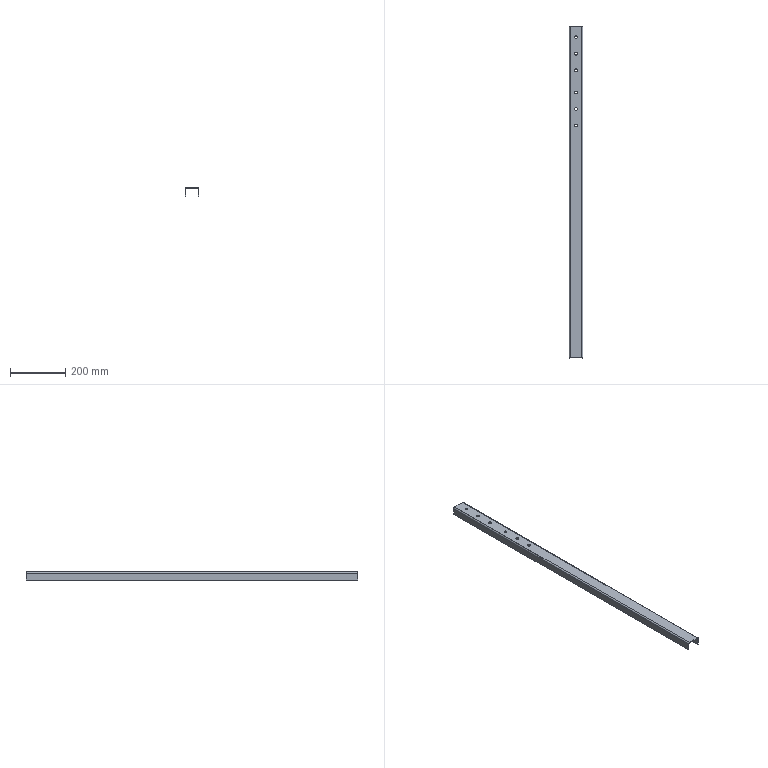Component | SolidWorks | 50x30x2ColdBentEqualAngleSteel1000mm-1 | 1 solid | 26 faces | box 50 x 1200 x 30 mm | volume 245217 mm3 | cylinder 16 | plane 10 | commonest cylinder face diameters 10 x14 6 x2
build123d program:
from build123d import *

# Parameters (mm, degrees)
BOSS_EXTRUDE1_DEPTH = 1200
SKETCH2_R           = 5
CUT_EXTRUDE1_DEPTH  = 207


with BuildPart() as part:
    # Sketch1 → Boss-Extrude1 (new body)
    with BuildSketch(Plane(origin=(0, 0, 0), x_dir=(0, 0, -1), z_dir=(1, 0, 0))):
        with BuildLine():
            Line((0, 5), (0, 45))
            ThreePointArc((0, 45), (1.464, 48.536), (5, 50))
            Line((5, 50), (30, 50))
            Line((30, 50), (30, 48))
            Line((30, 48), (5, 48))
            ThreePointArc((5, 48), (2.879, 47.121), (2, 45))
            Line((2, 45), (2, 5))
            ThreePointArc((2, 5), (2.879, 2.879), (5, 2))
            Line((5, 2), (30, 2))
            Line((30, 2), (30, 0))
            Line((30, 0), (5, 0))
            ThreePointArc((5, 0), (1.464, 1.464), (0, 5))
        make_face()
    extrude(amount=BOSS_EXTRUDE1_DEPTH)

    # Sketch2 → Cut-Extrude1 (cut)
    with BuildSketch(Plane.XY):
        with Locations((40, 25)):
            Circle(SKETCH2_R)
        with Locations((100, 25)):
            Circle(SKETCH2_R)
        with Locations((160, 25)):
            Circle(SKETCH2_R)
        with Locations((240, 25)):
            Circle(SKETCH2_R)
        with Locations((300, 25)):
            Circle(SKETCH2_R)
        with Locations((360, 25)):
            Circle(SKETCH2_R)
    extrude(amount=-CUT_EXTRUDE1_DEPTH, mode=Mode.SUBTRACT)


solid = part.part

# Placed as in the assembly
solid = solid.moved(Location((-624.371, -247.9, 415), (0, 0, -90)))
STEP:
#1=CARTESIAN_POINT('',(-23.597,-11.138,16.26));
#2=VERTEX_POINT('',#1);
#3=CARTESIAN_POINT('',(-23.597,-11.532,16.26));
#4=VERTEX_POINT('',#3);
#5=CARTESIAN_POINT('',(-23.597,-11.335,16.26));
#6=DIRECTION('',(-0.,-0.,1.));
#7=DIRECTION('',(0.,-1.,0.));
#8=AXIS2_PLACEMENT_3D('',#5,#6,#7);
#9=CIRCLE('',#8,0.1969);
#10=EDGE_CURVE('',#2,#4,#9,.T.);
#11=ORIENTED_EDGE('',*,*,#10,.F.);
#12=CARTESIAN_POINT('',(-23.597,-11.138,16.339));
#13=VERTEX_POINT('',#12);
#14=CARTESIAN_POINT('',(-23.597,-11.138,8.189));
#15=DIRECTION('',(-0.,-0.,1.));
#16=VECTOR('',#15,39.37);
#17=LINE('',#14,#16);
#18=EDGE_CURVE('',#2,#13,#17,.T.);
#19=ORIENTED_EDGE('',*,*,#18,.T.);
#20=CARTESIAN_POINT('',(-23.597,-11.532,16.339));
#21=VERTEX_POINT('',#20);
#22=CARTESIAN_POINT('',(-23.597,-11.335,16.339));
#23=DIRECTION('',(-0.,-0.,1.));
#24=DIRECTION('',(0.,-1.,0.));
#25=AXIS2_PLACEMENT_3D('',#22,#23,#24);
#26=CIRCLE('',#25,0.1969);
#27=EDGE_CURVE('',#13,#21,#26,.T.);
#28=ORIENTED_EDGE('',*,*,#27,.T.);
#29=CARTESIAN_POINT('',(-23.597,-11.532,8.189));
#30=DIRECTION('',(-0.,-0.,1.));
#31=VECTOR('',#30,39.37);
#32=LINE('',#29,#31);
#33=EDGE_CURVE('',#4,#21,#32,.T.);
#34=ORIENTED_EDGE('',*,*,#33,.F.);
#35=EDGE_LOOP('',(#11,#19,#28,#34));
#36=FACE_OUTER_BOUND('',#35,.T.);
#37=CARTESIAN_POINT('',(-23.597,-11.335,8.189));
#38=DIRECTION('',(-0.,-0.,1.));
#39=DIRECTION('',(0.,-1.,0.));
#40=AXIS2_PLACEMENT_3D('',#37,#38,#39);
#41=CYLINDRICAL_SURFACE('',#40,0.1969);
#42=ADVANCED_FACE('',(#36),#41,.F.);
#43=CARTESIAN_POINT('',(-23.597,-13.5,16.26));
#44=VERTEX_POINT('',#43);
#45=CARTESIAN_POINT('',(-23.597,-13.894,16.26));
#46=VERTEX_POINT('',#45);
#47=CARTESIAN_POINT('',(-23.597,-13.697,16.26));
#48=DIRECTION('',(-0.,-0.,1.));
#49=DIRECTION('',(0.,-1.,0.));
#50=AXIS2_PLACEMENT_3D('',#47,#48,#49);
#51=CIRCLE('',#50,0.1969);
#52=EDGE_CURVE('',#44,#46,#51,.T.);
#53=ORIENTED_EDGE('',*,*,#52,.F.);
#54=CARTESIAN_POINT('',(-23.597,-13.5,16.339));
#55=VERTEX_POINT('',#54);
#56=CARTESIAN_POINT('',(-23.597,-13.5,8.189));
#57=DIRECTION('',(-0.,-0.,1.));
#58=VECTOR('',#57,39.37);
#59=LINE('',#56,#58);
#60=EDGE_CURVE('',#44,#55,#59,.T.);
#61=ORIENTED_EDGE('',*,*,#60,.T.);
#62=CARTESIAN_POINT('',(-23.597,-13.894,16.339));
#63=VERTEX_POINT('',#62);
#64=CARTESIAN_POINT('',(-23.597,-13.697,16.339));
#65=DIRECTION('',(-0.,-0.,1.));
#66=DIRECTION('',(0.,-1.,0.));
#67=AXIS2_PLACEMENT_3D('',#64,#65,#66);
#68=CIRCLE('',#67,0.1969);
#69=EDGE_CURVE('',#55,#63,#68,.T.);
#70=ORIENTED_EDGE('',*,*,#69,.T.);
#71=CARTESIAN_POINT('',(-23.597,-13.894,8.189));
#72=DIRECTION('',(-0.,-0.,1.));
#73=VECTOR('',#72,39.37);
#74=LINE('',#71,#73);
#75=EDGE_CURVE('',#46,#63,#74,.T.);
#76=ORIENTED_EDGE('',*,*,#75,.F.);
#77=EDGE_LOOP('',(#53,#61,#70,#76));
#78=FACE_OUTER_BOUND('',#77,.T.);
#79=CARTESIAN_POINT('',(-23.597,-13.697,8.189));
#80=DIRECTION('',(-0.,-0.,1.));
#81=DIRECTION('',(0.,-1.,0.));
#82=AXIS2_PLACEMENT_3D('',#79,#80,#81);
#83=CYLINDRICAL_SURFACE('',#82,0.1969);
#84=ADVANCED_FACE('',(#78),#83,.F.);
#85=CARTESIAN_POINT('',(-23.597,-15.862,16.26));
#86=VERTEX_POINT('',#85);
#87=CARTESIAN_POINT('',(-23.597,-16.256,16.26));
#88=VERTEX_POINT('',#87);
#89=CARTESIAN_POINT('',(-23.597,-16.059,16.26));
#90=DIRECTION('',(-0.,-0.,1.));
#91=DIRECTION('',(0.,-1.,0.));
#92=AXIS2_PLACEMENT_3D('',#89,#90,#91);
#93=CIRCLE('',#92,0.1969);
#94=EDGE_CURVE('',#86,#88,#93,.T.);
#95=ORIENTED_EDGE('',*,*,#94,.F.);
#96=CARTESIAN_POINT('',(-23.597,-15.862,16.339));
#97=VERTEX_POINT('',#96);
#98=CARTESIAN_POINT('',(-23.597,-15.862,8.189));
#99=DIRECTION('',(-0.,-0.,1.));
#100=VECTOR('',#99,39.37);
#101=LINE('',#98,#100);
#102=EDGE_CURVE('',#86,#97,#101,.T.);
#103=ORIENTED_EDGE('',*,*,#102,.T.);
#104=CARTESIAN_POINT('',(-23.597,-16.256,16.339));
#105=VERTEX_POINT('',#104);
#106=CARTESIAN_POINT('',(-23.597,-16.059,16.339));
#107=DIRECTION('',(-0.,-0.,1.));
#108=DIRECTION('',(0.,-1.,0.));
#109=AXIS2_PLACEMENT_3D('',#106,#107,#108);
#110=CIRCLE('',#109,0.1969);
#111=EDGE_CURVE('',#97,#105,#110,.T.);
#112=ORIENTED_EDGE('',*,*,#111,.T.);
#113=CARTESIAN_POINT('',(-23.597,-16.256,8.189));
#114=DIRECTION('',(-0.,-0.,1.));
#115=VECTOR('',#114,39.37);
#116=LINE('',#113,#115);
#117=EDGE_CURVE('',#88,#105,#116,.T.);
#118=ORIENTED_EDGE('',*,*,#117,.F.);
#119=EDGE_LOOP('',(#95,#103,#112,#118));
#120=FACE_OUTER_BOUND('',#119,.T.);
#121=CARTESIAN_POINT('',(-23.597,-16.059,8.189));
#122=DIRECTION('',(-0.,-0.,1.));
#123=DIRECTION('',(0.,-1.,0.));
#124=AXIS2_PLACEMENT_3D('',#121,#122,#123);
#125=CYLINDRICAL_SURFACE('',#124,0.1969);
#126=ADVANCED_FACE('',(#120),#125,.F.);
#127=CARTESIAN_POINT('',(-23.597,-19.012,16.26));
#128=VERTEX_POINT('',#127);
#129=CARTESIAN_POINT('',(-23.597,-19.406,16.26));
#130=VERTEX_POINT('',#129);
#131=CARTESIAN_POINT('',(-23.597,-19.209,16.26));
#132=DIRECTION('',(-0.,-0.,1.));
#133=DIRECTION('',(0.,-1.,0.));
#134=AXIS2_PLACEMENT_3D('',#131,#132,#133);
#135=CIRCLE('',#134,0.1969);
#136=EDGE_CURVE('',#128,#130,#135,.T.);
#137=ORIENTED_EDGE('',*,*,#136,.F.);
#138=CARTESIAN_POINT('',(-23.597,-19.012,16.339));
#139=VERTEX_POINT('',#138);
#140=CARTESIAN_POINT('',(-23.597,-19.012,8.189));
#141=DIRECTION('',(-0.,-0.,1.));
#142=VECTOR('',#141,39.37);
#143=LINE('',#140,#142);
#144=EDGE_CURVE('',#128,#139,#143,.T.);
#145=ORIENTED_EDGE('',*,*,#144,.T.);
#146=CARTESIAN_POINT('',(-23.597,-19.406,16.339));
#147=VERTEX_POINT('',#146);
#148=CARTESIAN_POINT('',(-23.597,-19.209,16.339));
#149=DIRECTION('',(-0.,-0.,1.));
#150=DIRECTION('',(0.,-1.,0.));
#151=AXIS2_PLACEMENT_3D('',#148,#149,#150);
#152=CIRCLE('',#151,0.1969);
#153=EDGE_CURVE('',#139,#147,#152,.T.);
#154=ORIENTED_EDGE('',*,*,#153,.T.);
#155=CARTESIAN_POINT('',(-23.597,-19.406,8.189));
#156=DIRECTION('',(-0.,-0.,1.));
#157=VECTOR('',#156,39.37);
#158=LINE('',#155,#157);
#159=EDGE_CURVE('',#130,#147,#158,.T.);
#160=ORIENTED_EDGE('',*,*,#159,.F.);
#161=EDGE_LOOP('',(#137,#145,#154,#160));
#162=FACE_OUTER_BOUND('',#161,.T.);
#163=CARTESIAN_POINT('',(-23.597,-19.209,8.189));
#164=DIRECTION('',(-0.,-0.,1.));
#165=DIRECTION('',(0.,-1.,0.));
#166=AXIS2_PLACEMENT_3D('',#163,#164,#165);
#167=CYLINDRICAL_SURFACE('',#166,0.1969);
#168=ADVANCED_FACE('',(#162),#167,.F.);
#169=CARTESIAN_POINT('',(-23.597,-21.374,16.26));
#170=VERTEX_POINT('',#169);
#171=CARTESIAN_POINT('',(-23.597,-21.768,16.26));
#172=VERTEX_POINT('',#171);
#173=CARTESIAN_POINT('',(-23.597,-21.571,16.26));
#174=DIRECTION('',(-0.,-0.,1.));
#175=DIRECTION('',(0.,-1.,0.));
#176=AXIS2_PLACEMENT_3D('',#173,#174,#175);
#177=CIRCLE('',#176,0.1969);
#178=EDGE_CURVE('',#170,#172,#177,.T.);
#179=ORIENTED_EDGE('',*,*,#178,.F.);
#180=CARTESIAN_POINT('',(-23.597,-21.374,16.339));
#181=VERTEX_POINT('',#180);
#182=CARTESIAN_POINT('',(-23.597,-21.374,8.189));
#183=DIRECTION('',(-0.,-0.,1.));
#184=VECTOR('',#183,39.37);
#185=LINE('',#182,#184);
#186=EDGE_CURVE('',#170,#181,#185,.T.);
#187=ORIENTED_EDGE('',*,*,#186,.T.);
#188=CARTESIAN_POINT('',(-23.597,-21.768,16.339));
#189=VERTEX_POINT('',#188);
#190=CARTESIAN_POINT('',(-23.597,-21.571,16.339));
#191=DIRECTION('',(-0.,-0.,1.));
#192=DIRECTION('',(0.,-1.,0.));
#193=AXIS2_PLACEMENT_3D('',#190,#191,#192);
#194=CIRCLE('',#193,0.1969);
#195=EDGE_CURVE('',#181,#189,#194,.T.);
#196=ORIENTED_EDGE('',*,*,#195,.T.);
#197=CARTESIAN_POINT('',(-23.597,-21.768,8.189));
#198=DIRECTION('',(-0.,-0.,1.));
#199=VECTOR('',#198,39.37);
#200=LINE('',#197,#199);
#201=EDGE_CURVE('',#172,#189,#200,.T.);
#202=ORIENTED_EDGE('',*,*,#201,.F.);
#203=EDGE_LOOP('',(#179,#187,#196,#202));
#204=FACE_OUTER_BOUND('',#203,.T.);
#205=CARTESIAN_POINT('',(-23.597,-21.571,8.189));
#206=DIRECTION('',(-0.,-0.,1.));
#207=DIRECTION('',(0.,-1.,0.));
#208=AXIS2_PLACEMENT_3D('',#205,#206,#207);
#209=CYLINDRICAL_SURFACE('',#208,0.1969);
#210=ADVANCED_FACE('',(#204),#209,.F.);
#211=CARTESIAN_POINT('',(-23.597,-23.736,16.26));
#212=VERTEX_POINT('',#211);
#213=CARTESIAN_POINT('',(-23.597,-24.13,16.26));
#214=VERTEX_POINT('',#213);
#215=CARTESIAN_POINT('',(-23.597,-23.933,16.26));
#216=DIRECTION('',(-0.,-0.,1.));
#217=DIRECTION('',(0.,-1.,0.));
#218=AXIS2_PLACEMENT_3D('',#215,#216,#217);
#219=CIRCLE('',#218,0.1969);
#220=EDGE_CURVE('',#212,#214,#219,.T.);
#221=ORIENTED_EDGE('',*,*,#220,.F.);
#222=CARTESIAN_POINT('',(-23.597,-23.736,16.339));
#223=VERTEX_POINT('',#222);
#224=CARTESIAN_POINT('',(-23.597,-23.736,8.189));
#225=DIRECTION('',(-0.,-0.,1.));
#226=VECTOR('',#225,39.37);
#227=LINE('',#224,#226);
#228=EDGE_CURVE('',#212,#223,#227,.T.);
#229=ORIENTED_EDGE('',*,*,#228,.T.);
#230=CARTESIAN_POINT('',(-23.597,-24.13,16.339));
#231=VERTEX_POINT('',#230);
#232=CARTESIAN_POINT('',(-23.597,-23.933,16.339));
#233=DIRECTION('',(-0.,-0.,1.));
#234=DIRECTION('',(0.,-1.,0.));
#235=AXIS2_PLACEMENT_3D('',#232,#233,#234);
#236=CIRCLE('',#235,0.1969);
#237=EDGE_CURVE('',#223,#231,#236,.T.);
#238=ORIENTED_EDGE('',*,*,#237,.T.);
#239=CARTESIAN_POINT('',(-23.597,-24.13,8.189));
#240=DIRECTION('',(-0.,-0.,1.));
#241=VECTOR('',#240,39.37);
#242=LINE('',#239,#241);
#243=EDGE_CURVE('',#214,#231,#242,.T.);
#244=ORIENTED_EDGE('',*,*,#243,.F.);
#245=EDGE_LOOP('',(#221,#229,#238,#244));
#246=FACE_OUTER_BOUND('',#245,.T.);
#247=CARTESIAN_POINT('',(-23.597,-23.933,8.189));
#248=DIRECTION('',(-0.,-0.,1.));
#249=DIRECTION('',(0.,-1.,0.));
#250=AXIS2_PLACEMENT_3D('',#247,#248,#249);
#251=CYLINDRICAL_SURFACE('',#250,0.1969);
#252=ADVANCED_FACE('',(#246),#251,.F.);
#253=CARTESIAN_POINT('',(-22.613,-9.76,16.142));
#254=VERTEX_POINT('',#253);
#255=CARTESIAN_POINT('',(-22.81,-9.76,16.339));
#256=VERTEX_POINT('',#255);
#257=CARTESIAN_POINT('',(-22.81,-9.76,16.142));
#258=DIRECTION('',(0.,-1.,-0.));
#259=DIRECTION('',(0.,0.,1.));
#260=AXIS2_PLACEMENT_3D('',#257,#258,#259);
#261=CIRCLE('',#260,0.1969);
#262=EDGE_CURVE('',#254,#256,#261,.T.);
#263=ORIENTED_EDGE('',*,*,#262,.T.);
#264=CARTESIAN_POINT('',(-22.81,-57.004,16.339));
#265=VERTEX_POINT('',#264);
#266=CARTESIAN_POINT('',(-22.81,-57.004,16.339));
#267=DIRECTION('',(-0.,1.,0.));
#268=VECTOR('',#267,39.37);
#269=LINE('',#266,#268);
#270=EDGE_CURVE('',#265,#256,#269,.T.);
#271=ORIENTED_EDGE('',*,*,#270,.F.);
#272=CARTESIAN_POINT('',(-22.613,-57.004,16.142));
#273=VERTEX_POINT('',#272);
#274=CARTESIAN_POINT('',(-22.81,-57.004,16.142));
#275=DIRECTION('',(0.,-1.,-0.));
#276=DIRECTION('',(0.,0.,1.));
#277=AXIS2_PLACEMENT_3D('',#274,#275,#276);
#278=CIRCLE('',#277,0.1969);
#279=EDGE_CURVE('',#273,#265,#278,.T.);
#280=ORIENTED_EDGE('',*,*,#279,.F.);
#281=CARTESIAN_POINT('',(-22.613,-57.004,16.142));
#282=DIRECTION('',(-0.,1.,0.));
#283=VECTOR('',#282,39.37);
#284=LINE('',#281,#283);
#285=EDGE_CURVE('',#273,#254,#284,.T.);
#286=ORIENTED_EDGE('',*,*,#285,.T.);
#287=EDGE_LOOP('',(#263,#271,#280,#286));
#288=FACE_OUTER_BOUND('',#287,.T.);
#289=CARTESIAN_POINT('',(-22.81,-57.004,16.142));
#290=DIRECTION('',(-0.,1.,0.));
#291=DIRECTION('',(0.,0.,1.));
#292=AXIS2_PLACEMENT_3D('',#289,#290,#291);
#293=CYLINDRICAL_SURFACE('',#292,0.1969);
#294=ADVANCED_FACE('',(#288),#293,.T.);
#295=CARTESIAN_POINT('',(-23.597,-11.335,16.339));
#296=DIRECTION('',(-0.,-0.,1.));
#297=DIRECTION('',(0.,-1.,0.));
#298=AXIS2_PLACEMENT_3D('',#295,#296,#297);
#299=CIRCLE('',#298,0.1969);
#300=EDGE_CURVE('',#21,#13,#299,.T.);
#301=ORIENTED_EDGE('',*,*,#300,.F.);
#302=ORIENTED_EDGE('',*,*,#27,.F.);
#303=EDGE_LOOP('',(#301,#302));
#304=FACE_BOUND('',#303,.T.);
#305=CARTESIAN_POINT('',(-23.597,-13.697,16.339));
#306=DIRECTION('',(-0.,-0.,1.));
#307=DIRECTION('',(0.,-1.,0.));
#308=AXIS2_PLACEMENT_3D('',#305,#306,#307);
#309=CIRCLE('',#308,0.1969);
#310=EDGE_CURVE('',#63,#55,#309,.T.);
#311=ORIENTED_EDGE('',*,*,#310,.F.);
#312=ORIENTED_EDGE('',*,*,#69,.F.);
#313=EDGE_LOOP('',(#311,#312));
#314=FACE_BOUND('',#313,.T.);
#315=CARTESIAN_POINT('',(-23.597,-16.059,16.339));
#316=DIRECTION('',(-0.,-0.,1.));
#317=DIRECTION('',(0.,-1.,0.));
#318=AXIS2_PLACEMENT_3D('',#315,#316,#317);
#319=CIRCLE('',#318,0.1969);
#320=EDGE_CURVE('',#105,#97,#319,.T.);
#321=ORIENTED_EDGE('',*,*,#320,.F.);
#322=ORIENTED_EDGE('',*,*,#111,.F.);
#323=EDGE_LOOP('',(#321,#322));
#324=FACE_BOUND('',#323,.T.);
#325=CARTESIAN_POINT('',(-23.597,-19.209,16.339));
#326=DIRECTION('',(-0.,-0.,1.));
#327=DIRECTION('',(0.,-1.,0.));
#328=AXIS2_PLACEMENT_3D('',#325,#326,#327);
#329=CIRCLE('',#328,0.1969);
#330=EDGE_CURVE('',#147,#139,#329,.T.);
#331=ORIENTED_EDGE('',*,*,#330,.F.);
#332=ORIENTED_EDGE('',*,*,#153,.F.);
#333=EDGE_LOOP('',(#331,#332));
#334=FACE_BOUND('',#333,.T.);
#335=CARTESIAN_POINT('',(-23.597,-21.571,16.339));
#336=DIRECTION('',(-0.,-0.,1.));
#337=DIRECTION('',(0.,-1.,0.));
#338=AXIS2_PLACEMENT_3D('',#335,#336,#337);
#339=CIRCLE('',#338,0.1969);
#340=EDGE_CURVE('',#189,#181,#339,.T.);
#341=ORIENTED_EDGE('',*,*,#340,.F.);
#342=ORIENTED_EDGE('',*,*,#195,.F.);
#343=EDGE_LOOP('',(#341,#342));
#344=FACE_BOUND('',#343,.T.);
#345=CARTESIAN_POINT('',(-23.597,-23.933,16.339));
#346=DIRECTION('',(-0.,-0.,1.));
#347=DIRECTION('',(0.,-1.,0.));
#348=AXIS2_PLACEMENT_3D('',#345,#346,#347);
#349=CIRCLE('',#348,0.1969);
#350=EDGE_CURVE('',#231,#223,#349,.T.);
#351=ORIENTED_EDGE('',*,*,#350,.F.);
#352=ORIENTED_EDGE('',*,*,#237,.F.);
#353=EDGE_LOOP('',(#351,#352));
#354=FACE_BOUND('',#353,.T.);
#355=CARTESIAN_POINT('',(-24.385,-9.76,16.339));
#356=VERTEX_POINT('',#355);
#357=CARTESIAN_POINT('',(-24.385,-9.76,16.339));
#358=DIRECTION('',(-1.,-0.,-0.));
#359=VECTOR('',#358,39.37);
#360=LINE('',#357,#359);
#361=EDGE_CURVE('',#256,#356,#360,.T.);
#362=ORIENTED_EDGE('',*,*,#361,.T.);
#363=CARTESIAN_POINT('',(-24.385,-57.004,16.339));
#364=VERTEX_POINT('',#363);
#365=CARTESIAN_POINT('',(-24.385,-57.004,16.339));
#366=DIRECTION('',(-0.,1.,0.));
#367=VECTOR('',#366,39.37);
#368=LINE('',#365,#367);
#369=EDGE_CURVE('',#364,#356,#368,.T.);
#370=ORIENTED_EDGE('',*,*,#369,.F.);
#371=CARTESIAN_POINT('',(-24.385,-57.004,16.339));
#372=DIRECTION('',(-1.,-0.,-0.));
#373=VECTOR('',#372,39.37);
#374=LINE('',#371,#373);
#375=EDGE_CURVE('',#265,#364,#374,.T.);
#376=ORIENTED_EDGE('',*,*,#375,.F.);
#377=ORIENTED_EDGE('',*,*,#270,.T.);
#378=EDGE_LOOP('',(#362,#370,#376,#377));
#379=FACE_OUTER_BOUND('',#378,.T.);
#380=CARTESIAN_POINT('',(-24.385,-57.004,16.339));
#381=DIRECTION('',(0.,0.,-1.));
#382=DIRECTION('',(-0.,1.,0.));
#383=AXIS2_PLACEMENT_3D('',#380,#381,#382);
#384=PLANE('',#383);
#385=ADVANCED_FACE('',(#304,#314,#324,#334,#344,#354,#379),#384,.F.);
#386=CARTESIAN_POINT('',(-24.582,-9.76,16.142));
#387=VERTEX_POINT('',#386);
#388=CARTESIAN_POINT('',(-24.385,-9.76,16.142));
#389=DIRECTION('',(0.,-1.,-0.));
#390=DIRECTION('',(0.,0.,-1.));
#391=AXIS2_PLACEMENT_3D('',#388,#389,#390);
#392=CIRCLE('',#391,0.1969);
#393=EDGE_CURVE('',#356,#387,#392,.T.);
#394=ORIENTED_EDGE('',*,*,#393,.T.);
#395=CARTESIAN_POINT('',(-24.582,-57.004,16.142));
#396=VERTEX_POINT('',#395);
#397=CARTESIAN_POINT('',(-24.582,-57.004,16.142));
#398=DIRECTION('',(-0.,1.,0.));
#399=VECTOR('',#398,39.37);
#400=LINE('',#397,#399);
#401=EDGE_CURVE('',#396,#387,#400,.T.);
#402=ORIENTED_EDGE('',*,*,#401,.F.);
#403=CARTESIAN_POINT('',(-24.385,-57.004,16.142));
#404=DIRECTION('',(0.,-1.,-0.));
#405=DIRECTION('',(0.,0.,-1.));
#406=AXIS2_PLACEMENT_3D('',#403,#404,#405);
#407=CIRCLE('',#406,0.1969);
#408=EDGE_CURVE('',#364,#396,#407,.T.);
#409=ORIENTED_EDGE('',*,*,#408,.F.);
#410=ORIENTED_EDGE('',*,*,#369,.T.);
#411=EDGE_LOOP('',(#394,#402,#409,#410));
#412=FACE_OUTER_BOUND('',#411,.T.);
#413=CARTESIAN_POINT('',(-24.385,-57.004,16.142));
#414=DIRECTION('',(-0.,1.,0.));
#415=DIRECTION('',(0.,0.,1.));
#416=AXIS2_PLACEMENT_3D('',#413,#414,#415);
#417=CYLINDRICAL_SURFACE('',#416,0.1969);
#418=ADVANCED_FACE('',(#412),#417,.T.);
#419=CARTESIAN_POINT('',(-24.582,-9.76,15.157));
#420=VERTEX_POINT('',#419);
#421=CARTESIAN_POINT('',(-24.582,-9.76,16.142));
#422=DIRECTION('',(0.,0.,-1.));
#423=VECTOR('',#422,39.37);
#424=LINE('',#421,#423);
#425=EDGE_CURVE('',#387,#420,#424,.T.);
#426=ORIENTED_EDGE('',*,*,#425,.T.);
#427=CARTESIAN_POINT('',(-24.582,-57.004,15.157));
#428=VERTEX_POINT('',#427);
#429=CARTESIAN_POINT('',(-24.582,-57.004,15.157));
#430=DIRECTION('',(-0.,1.,0.));
#431=VECTOR('',#430,39.37);
#432=LINE('',#429,#431);
#433=EDGE_CURVE('',#428,#420,#432,.T.);
#434=ORIENTED_EDGE('',*,*,#433,.F.);
#435=CARTESIAN_POINT('',(-24.582,-57.004,16.142));
#436=DIRECTION('',(0.,0.,-1.));
#437=VECTOR('',#436,39.37);
#438=LINE('',#435,#437);
#439=EDGE_CURVE('',#396,#428,#438,.T.);
#440=ORIENTED_EDGE('',*,*,#439,.F.);
#441=ORIENTED_EDGE('',*,*,#401,.T.);
#442=EDGE_LOOP('',(#426,#434,#440,#441));
#443=FACE_OUTER_BOUND('',#442,.T.);
#444=CARTESIAN_POINT('',(-24.582,-57.004,16.142));
#445=DIRECTION('',(1.,0.,0.));
#446=DIRECTION('',(-0.,-0.,1.));
#447=AXIS2_PLACEMENT_3D('',#444,#445,#446);
#448=PLANE('',#447);
#449=ADVANCED_FACE('',(#443),#448,.F.);
#450=CARTESIAN_POINT('',(-24.503,-9.76,15.157));
#451=VERTEX_POINT('',#450);
#452=CARTESIAN_POINT('',(-24.503,-9.76,15.157));
#453=DIRECTION('',(1.,0.,0.));
#454=VECTOR('',#453,39.37);
#455=LINE('',#452,#454);
#456=EDGE_CURVE('',#420,#451,#455,.T.);
#457=ORIENTED_EDGE('',*,*,#456,.T.);
#458=CARTESIAN_POINT('',(-24.503,-57.004,15.157));
#459=VERTEX_POINT('',#458);
#460=CARTESIAN_POINT('',(-24.503,-57.004,15.157));
#461=DIRECTION('',(-0.,1.,0.));
#462=VECTOR('',#461,39.37);
#463=LINE('',#460,#462);
#464=EDGE_CURVE('',#459,#451,#463,.T.);
#465=ORIENTED_EDGE('',*,*,#464,.F.);
#466=CARTESIAN_POINT('',(-24.503,-57.004,15.157));
#467=DIRECTION('',(1.,0.,0.));
#468=VECTOR('',#467,39.37);
#469=LINE('',#466,#468);
#470=EDGE_CURVE('',#428,#459,#469,.T.);
#471=ORIENTED_EDGE('',*,*,#470,.F.);
#472=ORIENTED_EDGE('',*,*,#433,.T.);
#473=EDGE_LOOP('',(#457,#465,#471,#472));
#474=FACE_OUTER_BOUND('',#473,.T.);
#475=CARTESIAN_POINT('',(-24.503,-57.004,15.157));
#476=DIRECTION('',(-0.,-0.,1.));
#477=DIRECTION('',(0.,-1.,-0.));
#478=AXIS2_PLACEMENT_3D('',#475,#476,#477);
#479=PLANE('',#478);
#480=ADVANCED_FACE('',(#474),#479,.F.);
#481=CARTESIAN_POINT('',(-24.503,-9.76,16.142));
#482=VERTEX_POINT('',#481);
#483=CARTESIAN_POINT('',(-24.503,-9.76,16.142));
#484=DIRECTION('',(-0.,-0.,1.));
#485=VECTOR('',#484,39.37);
#486=LINE('',#483,#485);
#487=EDGE_CURVE('',#451,#482,#486,.T.);
#488=ORIENTED_EDGE('',*,*,#487,.T.);
#489=CARTESIAN_POINT('',(-24.503,-57.004,16.142));
#490=VERTEX_POINT('',#489);
#491=CARTESIAN_POINT('',(-24.503,-57.004,16.142));
#492=DIRECTION('',(-0.,1.,0.));
#493=VECTOR('',#492,39.37);
#494=LINE('',#491,#493);
#495=EDGE_CURVE('',#490,#482,#494,.T.);
#496=ORIENTED_EDGE('',*,*,#495,.F.);
#497=CARTESIAN_POINT('',(-24.503,-57.004,16.142));
#498=DIRECTION('',(-0.,-0.,1.));
#499=VECTOR('',#498,39.37);
#500=LINE('',#497,#499);
#501=EDGE_CURVE('',#459,#490,#500,.T.);
#502=ORIENTED_EDGE('',*,*,#501,.F.);
#503=ORIENTED_EDGE('',*,*,#464,.T.);
#504=EDGE_LOOP('',(#488,#496,#502,#503));
#505=FACE_OUTER_BOUND('',#504,.T.);
#506=CARTESIAN_POINT('',(-24.503,-57.004,16.142));
#507=DIRECTION('',(-1.,-0.,-0.));
#508=DIRECTION('',(0.,0.,-1.));
#509=AXIS2_PLACEMENT_3D('',#506,#507,#508);
#510=PLANE('',#509);
#511=ADVANCED_FACE('',(#505),#510,.F.);
#512=CARTESIAN_POINT('',(-24.385,-9.76,16.26));
#513=VERTEX_POINT('',#512);
#514=CARTESIAN_POINT('',(-24.385,-9.76,16.142));
#515=DIRECTION('',(-0.,1.,0.));
#516=DIRECTION('',(0.,0.,-1.));
#517=AXIS2_PLACEMENT_3D('',#514,#515,#516);
#518=CIRCLE('',#517,0.1181);
#519=EDGE_CURVE('',#482,#513,#518,.T.);
#520=ORIENTED_EDGE('',*,*,#519,.T.);
#521=CARTESIAN_POINT('',(-24.385,-57.004,16.26));
#522=VERTEX_POINT('',#521);
#523=CARTESIAN_POINT('',(-24.385,-57.004,16.26));
#524=DIRECTION('',(-0.,1.,0.));
#525=VECTOR('',#524,39.37);
#526=LINE('',#523,#525);
#527=EDGE_CURVE('',#522,#513,#526,.T.);
#528=ORIENTED_EDGE('',*,*,#527,.F.);
#529=CARTESIAN_POINT('',(-24.385,-57.004,16.142));
#530=DIRECTION('',(-0.,1.,0.));
#531=DIRECTION('',(0.,0.,-1.));
#532=AXIS2_PLACEMENT_3D('',#529,#530,#531);
#533=CIRCLE('',#532,0.1181);
#534=EDGE_CURVE('',#490,#522,#533,.T.);
#535=ORIENTED_EDGE('',*,*,#534,.F.);
#536=ORIENTED_EDGE('',*,*,#495,.T.);
#537=EDGE_LOOP('',(#520,#528,#535,#536));
#538=FACE_OUTER_BOUND('',#537,.T.);
#539=CARTESIAN_POINT('',(-24.385,-57.004,16.142));
#540=DIRECTION('',(-0.,1.,0.));
#541=DIRECTION('',(0.,0.,1.));
#542=AXIS2_PLACEMENT_3D('',#539,#540,#541);
#543=CYLINDRICAL_SURFACE('',#542,0.1181);
#544=ADVANCED_FACE('',(#538),#543,.F.);
#545=CARTESIAN_POINT('',(-23.597,-11.335,16.26));
#546=DIRECTION('',(-0.,-0.,1.));
#547=DIRECTION('',(0.,-1.,0.));
#548=AXIS2_PLACEMENT_3D('',#545,#546,#547);
#549=CIRCLE('',#548,0.1969);
#550=EDGE_CURVE('',#4,#2,#549,.T.);
#551=ORIENTED_EDGE('',*,*,#550,.T.);
#552=ORIENTED_EDGE('',*,*,#10,.T.);
#553=EDGE_LOOP('',(#551,#552));
#554=FACE_BOUND('',#553,.T.);
#555=CARTESIAN_POINT('',(-23.597,-13.697,16.26));
#556=DIRECTION('',(-0.,-0.,1.));
#557=DIRECTION('',(0.,-1.,0.));
#558=AXIS2_PLACEMENT_3D('',#555,#556,#557);
#559=CIRCLE('',#558,0.1969);
#560=EDGE_CURVE('',#46,#44,#559,.T.);
#561=ORIENTED_EDGE('',*,*,#560,.T.);
#562=ORIENTED_EDGE('',*,*,#52,.T.);
#563=EDGE_LOOP('',(#561,#562));
#564=FACE_BOUND('',#563,.T.);
#565=CARTESIAN_POINT('',(-23.597,-16.059,16.26));
#566=DIRECTION('',(-0.,-0.,1.));
#567=DIRECTION('',(0.,-1.,0.));
#568=AXIS2_PLACEMENT_3D('',#565,#566,#567);
#569=CIRCLE('',#568,0.1969);
#570=EDGE_CURVE('',#88,#86,#569,.T.);
#571=ORIENTED_EDGE('',*,*,#570,.T.);
#572=ORIENTED_EDGE('',*,*,#94,.T.);
#573=EDGE_LOOP('',(#571,#572));
#574=FACE_BOUND('',#573,.T.);
#575=CARTESIAN_POINT('',(-23.597,-19.209,16.26));
#576=DIRECTION('',(-0.,-0.,1.));
#577=DIRECTION('',(0.,-1.,0.));
#578=AXIS2_PLACEMENT_3D('',#575,#576,#577);
#579=CIRCLE('',#578,0.1969);
#580=EDGE_CURVE('',#130,#128,#579,.T.);
#581=ORIENTED_EDGE('',*,*,#580,.T.);
#582=ORIENTED_EDGE('',*,*,#136,.T.);
#583=EDGE_LOOP('',(#581,#582));
#584=FACE_BOUND('',#583,.T.);
#585=CARTESIAN_POINT('',(-23.597,-21.571,16.26));
#586=DIRECTION('',(-0.,-0.,1.));
#587=DIRECTION('',(0.,-1.,0.));
#588=AXIS2_PLACEMENT_3D('',#585,#586,#587);
#589=CIRCLE('',#588,0.1969);
#590=EDGE_CURVE('',#172,#170,#589,.T.);
#591=ORIENTED_EDGE('',*,*,#590,.T.);
#592=ORIENTED_EDGE('',*,*,#178,.T.);
#593=EDGE_LOOP('',(#591,#592));
#594=FACE_BOUND('',#593,.T.);
#595=CARTESIAN_POINT('',(-23.597,-23.933,16.26));
#596=DIRECTION('',(-0.,-0.,1.));
#597=DIRECTION('',(0.,-1.,0.));
#598=AXIS2_PLACEMENT_3D('',#595,#596,#597);
#599=CIRCLE('',#598,0.1969);
#600=EDGE_CURVE('',#214,#212,#599,.T.);
#601=ORIENTED_EDGE('',*,*,#600,.T.);
#602=ORIENTED_EDGE('',*,*,#220,.T.);
#603=EDGE_LOOP('',(#601,#602));
#604=FACE_BOUND('',#603,.T.);
#605=CARTESIAN_POINT('',(-22.81,-9.76,16.26));
#606=VERTEX_POINT('',#605);
#607=CARTESIAN_POINT('',(-24.385,-9.76,16.26));
#608=DIRECTION('',(1.,0.,0.));
#609=VECTOR('',#608,39.37);
#610=LINE('',#607,#609);
#611=EDGE_CURVE('',#513,#606,#610,.T.);
#612=ORIENTED_EDGE('',*,*,#611,.T.);
#613=CARTESIAN_POINT('',(-22.81,-57.004,16.26));
#614=VERTEX_POINT('',#613);
#615=CARTESIAN_POINT('',(-22.81,-57.004,16.26));
#616=DIRECTION('',(-0.,1.,0.));
#617=VECTOR('',#616,39.37);
#618=LINE('',#615,#617);
#619=EDGE_CURVE('',#614,#606,#618,.T.);
#620=ORIENTED_EDGE('',*,*,#619,.F.);
#621=CARTESIAN_POINT('',(-24.385,-57.004,16.26));
#622=DIRECTION('',(1.,0.,0.));
#623=VECTOR('',#622,39.37);
#624=LINE('',#621,#623);
#625=EDGE_CURVE('',#522,#614,#624,.T.);
#626=ORIENTED_EDGE('',*,*,#625,.F.);
#627=ORIENTED_EDGE('',*,*,#527,.T.);
#628=EDGE_LOOP('',(#612,#620,#626,#627));
#629=FACE_OUTER_BOUND('',#628,.T.);
#630=CARTESIAN_POINT('',(-24.385,-57.004,16.26));
#631=DIRECTION('',(-0.,-0.,1.));
#632=DIRECTION('',(0.,-1.,-0.));
#633=AXIS2_PLACEMENT_3D('',#630,#631,#632);
#634=PLANE('',#633);
#635=ADVANCED_FACE('',(#554,#564,#574,#584,#594,#604,#629),#634,.F.);
#636=CARTESIAN_POINT('',(-22.692,-9.76,16.142));
#637=VERTEX_POINT('',#636);
#638=CARTESIAN_POINT('',(-22.81,-9.76,16.142));
#639=DIRECTION('',(-0.,1.,0.));
#640=DIRECTION('',(0.,0.,1.));
#641=AXIS2_PLACEMENT_3D('',#638,#639,#640);
#642=CIRCLE('',#641,0.1181);
#643=EDGE_CURVE('',#606,#637,#642,.T.);
#644=ORIENTED_EDGE('',*,*,#643,.T.);
#645=CARTESIAN_POINT('',(-22.692,-57.004,16.142));
#646=VERTEX_POINT('',#645);
#647=CARTESIAN_POINT('',(-22.692,-57.004,16.142));
#648=DIRECTION('',(-0.,1.,0.));
#649=VECTOR('',#648,39.37);
#650=LINE('',#647,#649);
#651=EDGE_CURVE('',#646,#637,#650,.T.);
#652=ORIENTED_EDGE('',*,*,#651,.F.);
#653=CARTESIAN_POINT('',(-22.81,-57.004,16.142));
#654=DIRECTION('',(-0.,1.,0.));
#655=DIRECTION('',(0.,0.,1.));
#656=AXIS2_PLACEMENT_3D('',#653,#654,#655);
#657=CIRCLE('',#656,0.1181);
#658=EDGE_CURVE('',#614,#646,#657,.T.);
#659=ORIENTED_EDGE('',*,*,#658,.F.);
#660=ORIENTED_EDGE('',*,*,#619,.T.);
#661=EDGE_LOOP('',(#644,#652,#659,#660));
#662=FACE_OUTER_BOUND('',#661,.T.);
#663=CARTESIAN_POINT('',(-22.81,-57.004,16.142));
#664=DIRECTION('',(-0.,1.,0.));
#665=DIRECTION('',(0.,0.,1.));
#666=AXIS2_PLACEMENT_3D('',#663,#664,#665);
#667=CYLINDRICAL_SURFACE('',#666,0.1181);
#668=ADVANCED_FACE('',(#662),#667,.F.);
#669=CARTESIAN_POINT('',(-22.692,-9.76,15.157));
#670=VERTEX_POINT('',#669);
#671=CARTESIAN_POINT('',(-22.692,-9.76,16.142));
#672=DIRECTION('',(0.,0.,-1.));
#673=VECTOR('',#672,39.37);
#674=LINE('',#671,#673);
#675=EDGE_CURVE('',#637,#670,#674,.T.);
#676=ORIENTED_EDGE('',*,*,#675,.T.);
#677=CARTESIAN_POINT('',(-22.692,-57.004,15.157));
#678=VERTEX_POINT('',#677);
#679=CARTESIAN_POINT('',(-22.692,-57.004,15.157));
#680=DIRECTION('',(-0.,1.,0.));
#681=VECTOR('',#680,39.37);
#682=LINE('',#679,#681);
#683=EDGE_CURVE('',#678,#670,#682,.T.);
#684=ORIENTED_EDGE('',*,*,#683,.F.);
#685=CARTESIAN_POINT('',(-22.692,-57.004,16.142));
#686=DIRECTION('',(0.,0.,-1.));
#687=VECTOR('',#686,39.37);
#688=LINE('',#685,#687);
#689=EDGE_CURVE('',#646,#678,#688,.T.);
#690=ORIENTED_EDGE('',*,*,#689,.F.);
#691=ORIENTED_EDGE('',*,*,#651,.T.);
#692=EDGE_LOOP('',(#676,#684,#690,#691));
#693=FACE_OUTER_BOUND('',#692,.T.);
#694=CARTESIAN_POINT('',(-22.692,-57.004,16.142));
#695=DIRECTION('',(1.,0.,0.));
#696=DIRECTION('',(-0.,-0.,1.));
#697=AXIS2_PLACEMENT_3D('',#694,#695,#696);
#698=PLANE('',#697);
#699=ADVANCED_FACE('',(#693),#698,.F.);
#700=CARTESIAN_POINT('',(-22.613,-9.76,15.157));
#701=VERTEX_POINT('',#700);
#702=CARTESIAN_POINT('',(-22.613,-9.76,15.157));
#703=DIRECTION('',(1.,0.,0.));
#704=VECTOR('',#703,39.37);
#705=LINE('',#702,#704);
#706=EDGE_CURVE('',#670,#701,#705,.T.);
#707=ORIENTED_EDGE('',*,*,#706,.T.);
#708=CARTESIAN_POINT('',(-22.613,-57.004,15.157));
#709=VERTEX_POINT('',#708);
#710=CARTESIAN_POINT('',(-22.613,-57.004,15.157));
#711=DIRECTION('',(-0.,1.,0.));
#712=VECTOR('',#711,39.37);
#713=LINE('',#710,#712);
#714=EDGE_CURVE('',#709,#701,#713,.T.);
#715=ORIENTED_EDGE('',*,*,#714,.F.);
#716=CARTESIAN_POINT('',(-22.613,-57.004,15.157));
#717=DIRECTION('',(1.,0.,0.));
#718=VECTOR('',#717,39.37);
#719=LINE('',#716,#718);
#720=EDGE_CURVE('',#678,#709,#719,.T.);
#721=ORIENTED_EDGE('',*,*,#720,.F.);
#722=ORIENTED_EDGE('',*,*,#683,.T.);
#723=EDGE_LOOP('',(#707,#715,#721,#722));
#724=FACE_OUTER_BOUND('',#723,.T.);
#725=CARTESIAN_POINT('',(-22.613,-57.004,15.157));
#726=DIRECTION('',(-0.,-0.,1.));
#727=DIRECTION('',(0.,-1.,-0.));
#728=AXIS2_PLACEMENT_3D('',#725,#726,#727);
#729=PLANE('',#728);
#730=ADVANCED_FACE('',(#724),#729,.F.);
#731=CARTESIAN_POINT('',(-22.613,-9.76,16.142));
#732=DIRECTION('',(-0.,-0.,1.));
#733=VECTOR('',#732,39.37);
#734=LINE('',#731,#733);
#735=EDGE_CURVE('',#701,#254,#734,.T.);
#736=ORIENTED_EDGE('',*,*,#735,.T.);
#737=ORIENTED_EDGE('',*,*,#285,.F.);
#738=CARTESIAN_POINT('',(-22.613,-57.004,16.142));
#739=DIRECTION('',(-0.,-0.,1.));
#740=VECTOR('',#739,39.37);
#741=LINE('',#738,#740);
#742=EDGE_CURVE('',#709,#273,#741,.T.);
#743=ORIENTED_EDGE('',*,*,#742,.F.);
#744=ORIENTED_EDGE('',*,*,#714,.T.);
#745=EDGE_LOOP('',(#736,#737,#743,#744));
#746=FACE_OUTER_BOUND('',#745,.T.);
#747=CARTESIAN_POINT('',(-22.613,-57.004,16.142));
#748=DIRECTION('',(-1.,-0.,-0.));
#749=DIRECTION('',(0.,0.,-1.));
#750=AXIS2_PLACEMENT_3D('',#747,#748,#749);
#751=PLANE('',#750);
#752=ADVANCED_FACE('',(#746),#751,.F.);
#753=ORIENTED_EDGE('',*,*,#279,.T.);
#754=ORIENTED_EDGE('',*,*,#375,.T.);
#755=ORIENTED_EDGE('',*,*,#408,.T.);
#756=ORIENTED_EDGE('',*,*,#439,.T.);
#757=ORIENTED_EDGE('',*,*,#470,.T.);
#758=ORIENTED_EDGE('',*,*,#501,.T.);
#759=ORIENTED_EDGE('',*,*,#534,.T.);
#760=ORIENTED_EDGE('',*,*,#625,.T.);
#761=ORIENTED_EDGE('',*,*,#658,.T.);
#762=ORIENTED_EDGE('',*,*,#689,.T.);
#763=ORIENTED_EDGE('',*,*,#720,.T.);
#764=ORIENTED_EDGE('',*,*,#742,.T.);
#765=EDGE_LOOP('',(#753,#754,#755,#756,#757,#758,#759,#760,#761,#762,#763,#764));
#766=FACE_OUTER_BOUND('',#765,.T.);
#767=CARTESIAN_POINT('',(-22.81,-57.004,16.142));
#768=DIRECTION('',(-0.,1.,0.));
#769=DIRECTION('',(-0.,-0.,1.));
#770=AXIS2_PLACEMENT_3D('',#767,#768,#769);
#771=PLANE('',#770);
#772=ADVANCED_FACE('',(#766),#771,.F.);
#773=ORIENTED_EDGE('',*,*,#262,.F.);
#774=ORIENTED_EDGE('',*,*,#735,.F.);
#775=ORIENTED_EDGE('',*,*,#706,.F.);
#776=ORIENTED_EDGE('',*,*,#675,.F.);
#777=ORIENTED_EDGE('',*,*,#643,.F.);
#778=ORIENTED_EDGE('',*,*,#611,.F.);
#779=ORIENTED_EDGE('',*,*,#519,.F.);
#780=ORIENTED_EDGE('',*,*,#487,.F.);
#781=ORIENTED_EDGE('',*,*,#456,.F.);
#782=ORIENTED_EDGE('',*,*,#425,.F.);
#783=ORIENTED_EDGE('',*,*,#393,.F.);
#784=ORIENTED_EDGE('',*,*,#361,.F.);
#785=EDGE_LOOP('',(#773,#774,#775,#776,#777,#778,#779,#780,#781,#782,#783,#784));
#786=FACE_OUTER_BOUND('',#785,.T.);
#787=CARTESIAN_POINT('',(-22.81,-9.76,16.142));
#788=DIRECTION('',(-0.,1.,0.));
#789=DIRECTION('',(-0.,-0.,1.));
#790=AXIS2_PLACEMENT_3D('',#787,#788,#789);
#791=PLANE('',#790);
#792=ADVANCED_FACE('',(#786),#791,.T.);
#793=ORIENTED_EDGE('',*,*,#228,.F.);
#794=ORIENTED_EDGE('',*,*,#600,.F.);
#795=ORIENTED_EDGE('',*,*,#243,.T.);
#796=ORIENTED_EDGE('',*,*,#350,.T.);
#797=EDGE_LOOP('',(#793,#794,#795,#796));
#798=FACE_OUTER_BOUND('',#797,.T.);
#799=CARTESIAN_POINT('',(-23.597,-23.933,8.189));
#800=DIRECTION('',(-0.,-0.,1.));
#801=DIRECTION('',(0.,-1.,0.));
#802=AXIS2_PLACEMENT_3D('',#799,#800,#801);
#803=CYLINDRICAL_SURFACE('',#802,0.1969);
#804=ADVANCED_FACE('',(#798),#803,.F.);
#805=ORIENTED_EDGE('',*,*,#186,.F.);
#806=ORIENTED_EDGE('',*,*,#590,.F.);
#807=ORIENTED_EDGE('',*,*,#201,.T.);
#808=ORIENTED_EDGE('',*,*,#340,.T.);
#809=EDGE_LOOP('',(#805,#806,#807,#808));
#810=FACE_OUTER_BOUND('',#809,.T.);
#811=CARTESIAN_POINT('',(-23.597,-21.571,8.189));
#812=DIRECTION('',(-0.,-0.,1.));
#813=DIRECTION('',(0.,-1.,0.));
#814=AXIS2_PLACEMENT_3D('',#811,#812,#813);
#815=CYLINDRICAL_SURFACE('',#814,0.1969);
#816=ADVANCED_FACE('',(#810),#815,.F.);
#817=ORIENTED_EDGE('',*,*,#144,.F.);
#818=ORIENTED_EDGE('',*,*,#580,.F.);
#819=ORIENTED_EDGE('',*,*,#159,.T.);
#820=ORIENTED_EDGE('',*,*,#330,.T.);
#821=EDGE_LOOP('',(#817,#818,#819,#820));
#822=FACE_OUTER_BOUND('',#821,.T.);
#823=CARTESIAN_POINT('',(-23.597,-19.209,8.189));
#824=DIRECTION('',(-0.,-0.,1.));
#825=DIRECTION('',(0.,-1.,0.));
#826=AXIS2_PLACEMENT_3D('',#823,#824,#825);
#827=CYLINDRICAL_SURFACE('',#826,0.1969);
#828=ADVANCED_FACE('',(#822),#827,.F.);
#829=ORIENTED_EDGE('',*,*,#102,.F.);
#830=ORIENTED_EDGE('',*,*,#570,.F.);
#831=ORIENTED_EDGE('',*,*,#117,.T.);
#832=ORIENTED_EDGE('',*,*,#320,.T.);
#833=EDGE_LOOP('',(#829,#830,#831,#832));
#834=FACE_OUTER_BOUND('',#833,.T.);
#835=CARTESIAN_POINT('',(-23.597,-16.059,8.189));
#836=DIRECTION('',(-0.,-0.,1.));
#837=DIRECTION('',(0.,-1.,0.));
#838=AXIS2_PLACEMENT_3D('',#835,#836,#837);
#839=CYLINDRICAL_SURFACE('',#838,0.1969);
#840=ADVANCED_FACE('',(#834),#839,.F.);
#841=ORIENTED_EDGE('',*,*,#60,.F.);
#842=ORIENTED_EDGE('',*,*,#560,.F.);
#843=ORIENTED_EDGE('',*,*,#75,.T.);
#844=ORIENTED_EDGE('',*,*,#310,.T.);
#845=EDGE_LOOP('',(#841,#842,#843,#844));
#846=FACE_OUTER_BOUND('',#845,.T.);
#847=CARTESIAN_POINT('',(-23.597,-13.697,8.189));
#848=DIRECTION('',(-0.,-0.,1.));
#849=DIRECTION('',(0.,-1.,0.));
#850=AXIS2_PLACEMENT_3D('',#847,#848,#849);
#851=CYLINDRICAL_SURFACE('',#850,0.1969);
#852=ADVANCED_FACE('',(#846),#851,.F.);
#853=ORIENTED_EDGE('',*,*,#18,.F.);
#854=ORIENTED_EDGE('',*,*,#550,.F.);
#855=ORIENTED_EDGE('',*,*,#33,.T.);
#856=ORIENTED_EDGE('',*,*,#300,.T.);
#857=EDGE_LOOP('',(#853,#854,#855,#856));
#858=FACE_OUTER_BOUND('',#857,.T.);
#859=CARTESIAN_POINT('',(-23.597,-11.335,8.189));
#860=DIRECTION('',(-0.,-0.,1.));
#861=DIRECTION('',(0.,-1.,0.));
#862=AXIS2_PLACEMENT_3D('',#859,#860,#861);
#863=CYLINDRICAL_SURFACE('',#862,0.1969);
#864=ADVANCED_FACE('',(#858),#863,.F.);
#865=CLOSED_SHELL('',(#42,#84,#126,#168,#210,#252,#294,#385,#418,#449,#480,#511,#544,#635,#668,#699,#730,#752,#772,#792,#804,#816,#828,#840,#852,#864));
#866=MANIFOLD_SOLID_BREP('',#865);
#867=CARTESIAN_POINT('',(0.,0.,0.));
#868=DIRECTION('',(0.,0.,1.));
#869=DIRECTION('',(1.,0.,0.));
#870=AXIS2_PLACEMENT_3D('',#867,#868,#869);
#871=(LENGTH_UNIT()NAMED_UNIT(*)SI_UNIT($,.METRE.));
#872=LENGTH_MEASURE_WITH_UNIT(LENGTH_MEASURE(0.0254),#871);
#873=DIMENSIONAL_EXPONENTS(1.,0.,0.,0.,0.,0.,0.);
#874=(CONVERSION_BASED_UNIT('',#872)LENGTH_UNIT()NAMED_UNIT(#873));
#875=UNCERTAINTY_MEASURE_WITH_UNIT(LENGTH_MEASURE(0.00001),#874,'','');
#876=(NAMED_UNIT(*)PLANE_ANGLE_UNIT()SI_UNIT($,.RADIAN.));
#877=(NAMED_UNIT(*)SI_UNIT($,.STERADIAN.)SOLID_ANGLE_UNIT());
#878=(GEOMETRIC_REPRESENTATION_CONTEXT(3)GLOBAL_UNCERTAINTY_ASSIGNED_CONTEXT((#875))GLOBAL_UNIT_ASSIGNED_CONTEXT((#874,#876,#877))REPRESENTATION_CONTEXT('',''));
#879=ADVANCED_BREP_SHAPE_REPRESENTATION('',(#866,#870),#878);
#880=COLOUR_RGB('',0.7922,0.8196,0.9333);
#881=FILL_AREA_STYLE_COLOUR('',#880);
#882=FILL_AREA_STYLE('',(#881));
#883=SURFACE_STYLE_FILL_AREA(#882);
#884=SURFACE_SIDE_STYLE('',(#883));
#885=SURFACE_STYLE_USAGE(.BOTH.,#884);
#886=PRESENTATION_STYLE_ASSIGNMENT((#885));
#887=STYLED_ITEM('',(#886),#866);
#888=PRESENTATION_LAYER_ASSIGNMENT('','',(#887));
#889=(LENGTH_UNIT()NAMED_UNIT(*)SI_UNIT($,.METRE.));
#890=LENGTH_MEASURE_WITH_UNIT(LENGTH_MEASURE(0.0254),#889);
#891=DIMENSIONAL_EXPONENTS(1.,0.,0.,0.,0.,0.,0.);
#892=(CONVERSION_BASED_UNIT('',#890)LENGTH_UNIT()NAMED_UNIT(#891));
#893=UNCERTAINTY_MEASURE_WITH_UNIT(LENGTH_MEASURE(0.00001),#892,'','');
#894=(NAMED_UNIT(*)PLANE_ANGLE_UNIT()SI_UNIT($,.RADIAN.));
#895=(NAMED_UNIT(*)SI_UNIT($,.STERADIAN.)SOLID_ANGLE_UNIT());
#896=(GEOMETRIC_REPRESENTATION_CONTEXT(3)GLOBAL_UNCERTAINTY_ASSIGNED_CONTEXT((#893))GLOBAL_UNIT_ASSIGNED_CONTEXT((#892,#894,#895))REPRESENTATION_CONTEXT('',''));
#897=MECHANICAL_DESIGN_GEOMETRIC_PRESENTATION_REPRESENTATION('',(#887),#896);